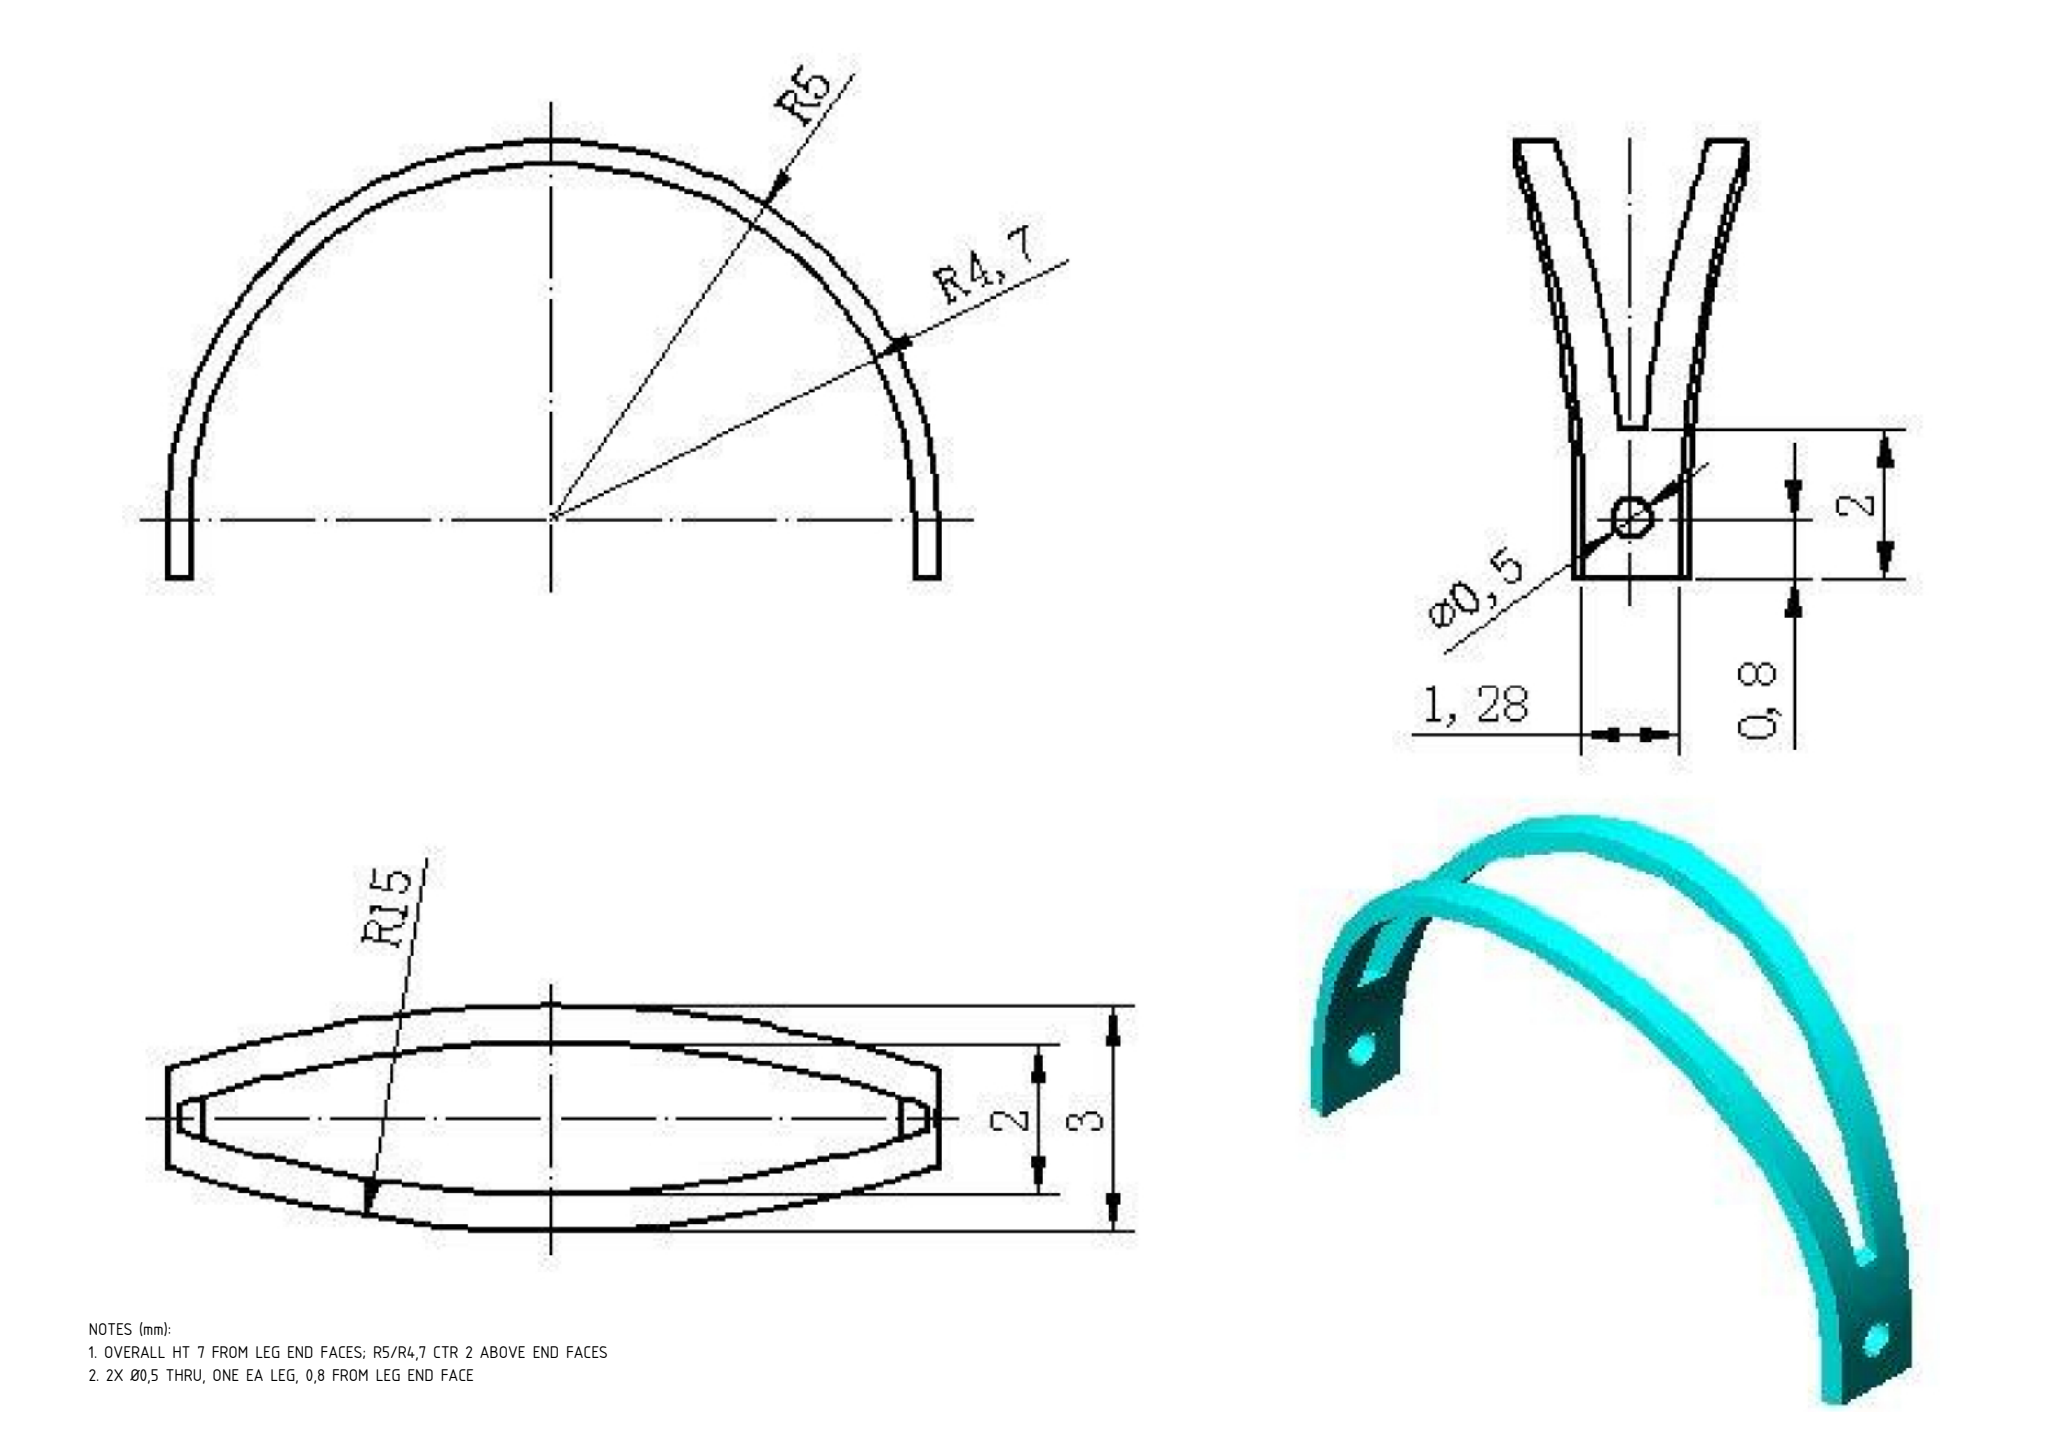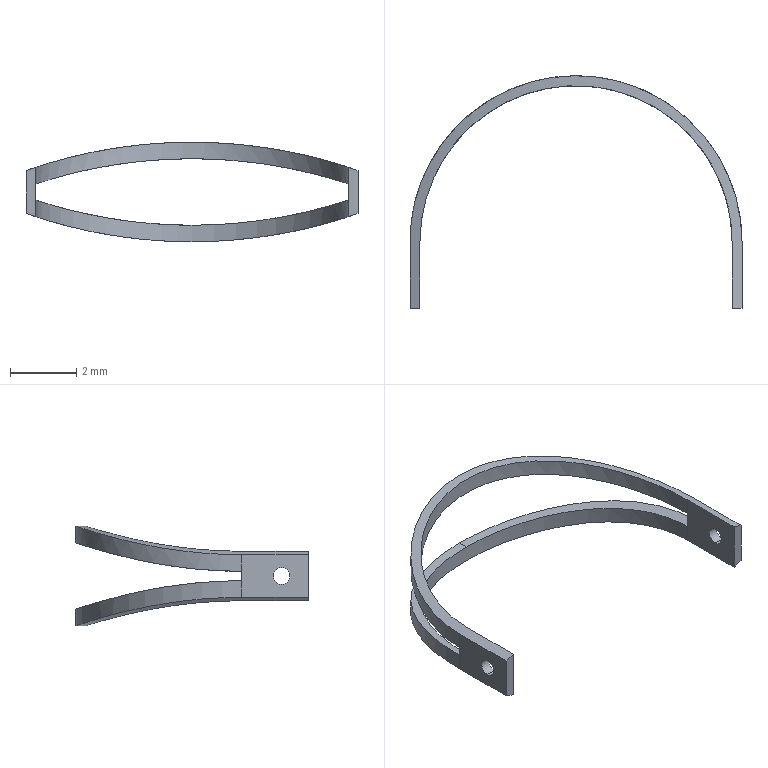Part | SolidWorks | mm | 1 solid | 22 faces | box 10 x 7 x 3 mm | volume 6 mm3 | cylinder 14 | plane 8 | commonest cylinder face diameters 30 x6 0.5 x4 10 x2 9.4 x2
Drawing notes:
OVERALL HT 7 FROM LEG END FACES; R5/R4,7 CTR 2 ABOVE END FACES | from the solid: bbox y=7.002; R5 & R4,7 arc cyls (dia 10/9.4, axis z) at y=2.0 from bbox min face
2X Ø0,5 THRU, ONE EA LEG, 0,8 FROM LEG END FACE | from the solid: 4 cyl faces dia 0.5, axis x, y=0.8, z=1.5, len 0.3 each thru 0.3 walls at x=0-0.3 and 9.7-10 = 2 holes
build123d program:
from build123d import *

# Parameters (mm, degrees)
BOSS_EXTRUDE1_DEPTH     = 1.5
CUT_EXTRUDE2_DEPTH      = 8.228
CUT_EXTRUDE2_DEPTH_BACK = 8.228
CUT_EXTRUDE4_DEPTH      = 8.228
BOSS_EXTRUDE4_START     = 1.2
BOSS_EXTRUDE4_DEPTH     = 1.2
CUT_EXTRUDE5_DEPTH      = 8.228
CUT_EXTRUDE5_DEPTH_BACK = 8.228
SKETCH7_R               = 0.25


with BuildPart() as part:
    # Sketch1 → Boss-Extrude1 (new, symmetric)
    with BuildSketch(Plane.XY):
        with BuildLine():
            Line((-5, 0), (-5, -0.8))
            Line((-5, -0.8), (-4.7, -0.8))
            Line((-4.7, -0.8), (-4.7, 0))
            ThreePointArc((-4.7, 0), (0, 4.7), (4.7, 0))
            Line((4.7, 0), (4.7, -0.8))
            Line((4.7, -0.8), (5, -0.8))
            Line((5, -0.8), (5, 0))
            ThreePointArc((5, 0), (0, 5), (-5, 0))
        make_face()
    extrude(amount=BOSS_EXTRUDE1_DEPTH, both=True)

    # Sketch2 → Cut-Extrude2 (cut, two sides: drawn at the far end of the back side and taken through both)
    with BuildSketch(Plane(origin=(0, 0, 0), x_dir=(1, 0, 0), z_dir=(0, 1, 0)).offset(-CUT_EXTRUDE2_DEPTH_BACK)):
        with BuildLine():
            Line((-5, 1.5), (-5, 0.6421))
            ThreePointArc((-5, 0.6421), (-2.537, 1.284), (0, 1.5))
            Line((0, 1.5), (-5, 1.5))
        make_face()
        with BuildLine():
            ThreePointArc((0, 1.5), (2.537, 1.284), (5, 0.6421))
            Line((5, 0.6421), (5, 1.5))
            Line((5, 1.5), (0, 1.5))
        make_face()
        with BuildLine():
            ThreePointArc((5, -0.6421), (2.537, -1.284), (0, -1.5))
            Line((0, -1.5), (5, -1.5))
            Line((5, -1.5), (5, -0.6421))
        make_face()
        with BuildLine():
            Line((-5, -0.6421), (-5, -1.5))
            Line((-5, -1.5), (0, -1.5))
            ThreePointArc((0, -1.5), (-2.537, -1.284), (-5, -0.6421))
        make_face()
    extrude(amount=CUT_EXTRUDE2_DEPTH + CUT_EXTRUDE2_DEPTH_BACK, mode=Mode.SUBTRACT)

    # Sketch3 → Cut-Extrude4 (cut, through all)
    with BuildSketch(Plane(origin=(0, 0, 0), x_dir=(1, 0, 0), z_dir=(0, 1, 0))):
        with BuildLine():
            ThreePointArc((5.385, 0), (0, 1), (-5.385, 0))
            ThreePointArc((-5.385, 0), (0, -1), (5.385, 0))
        make_face()
    extrude(amount=CUT_EXTRUDE4_DEPTH, mode=Mode.SUBTRACT)

    # Sketch6 → Boss-Extrude4 (add)
    with BuildSketch(Plane.XZ.offset(0.8).offset(BOSS_EXTRUDE4_START)):
        with BuildLine():
            Line((4.7, 0.7446), (4.7, -0.7446))
            ThreePointArc((4.7, -0.7446), (4.85, -0.6942), (5, -0.6421))
            Line((5, -0.6421), (5, 0.6421))
            ThreePointArc((5, 0.6421), (4.85, 0.6942), (4.7, 0.7446))
        make_face()
        with BuildLine():
            Line((-5, 0.6421), (-5, -0.6421))
            ThreePointArc((-5, -0.6421), (-4.85, -0.6942), (-4.7, -0.7446))
            Line((-4.7, -0.7446), (-4.7, 0.7446))
            ThreePointArc((-4.7, 0.7446), (-4.85, 0.6942), (-5, 0.6421))
        make_face()
    extrude(amount=-BOSS_EXTRUDE4_DEPTH)

    # Sketch7 → Cut-Extrude5 (cut, two sides: drawn at the far end of the back side and taken through both)
    with BuildSketch(Plane(origin=(0, 0, 0), x_dir=(0, 0, -1), z_dir=(1, 0, 0)).offset(-CUT_EXTRUDE5_DEPTH_BACK)):
        with Locations((0, -1.2)):
            Circle(SKETCH7_R)
    extrude(amount=CUT_EXTRUDE5_DEPTH + CUT_EXTRUDE5_DEPTH_BACK, mode=Mode.SUBTRACT)


solid = part.part